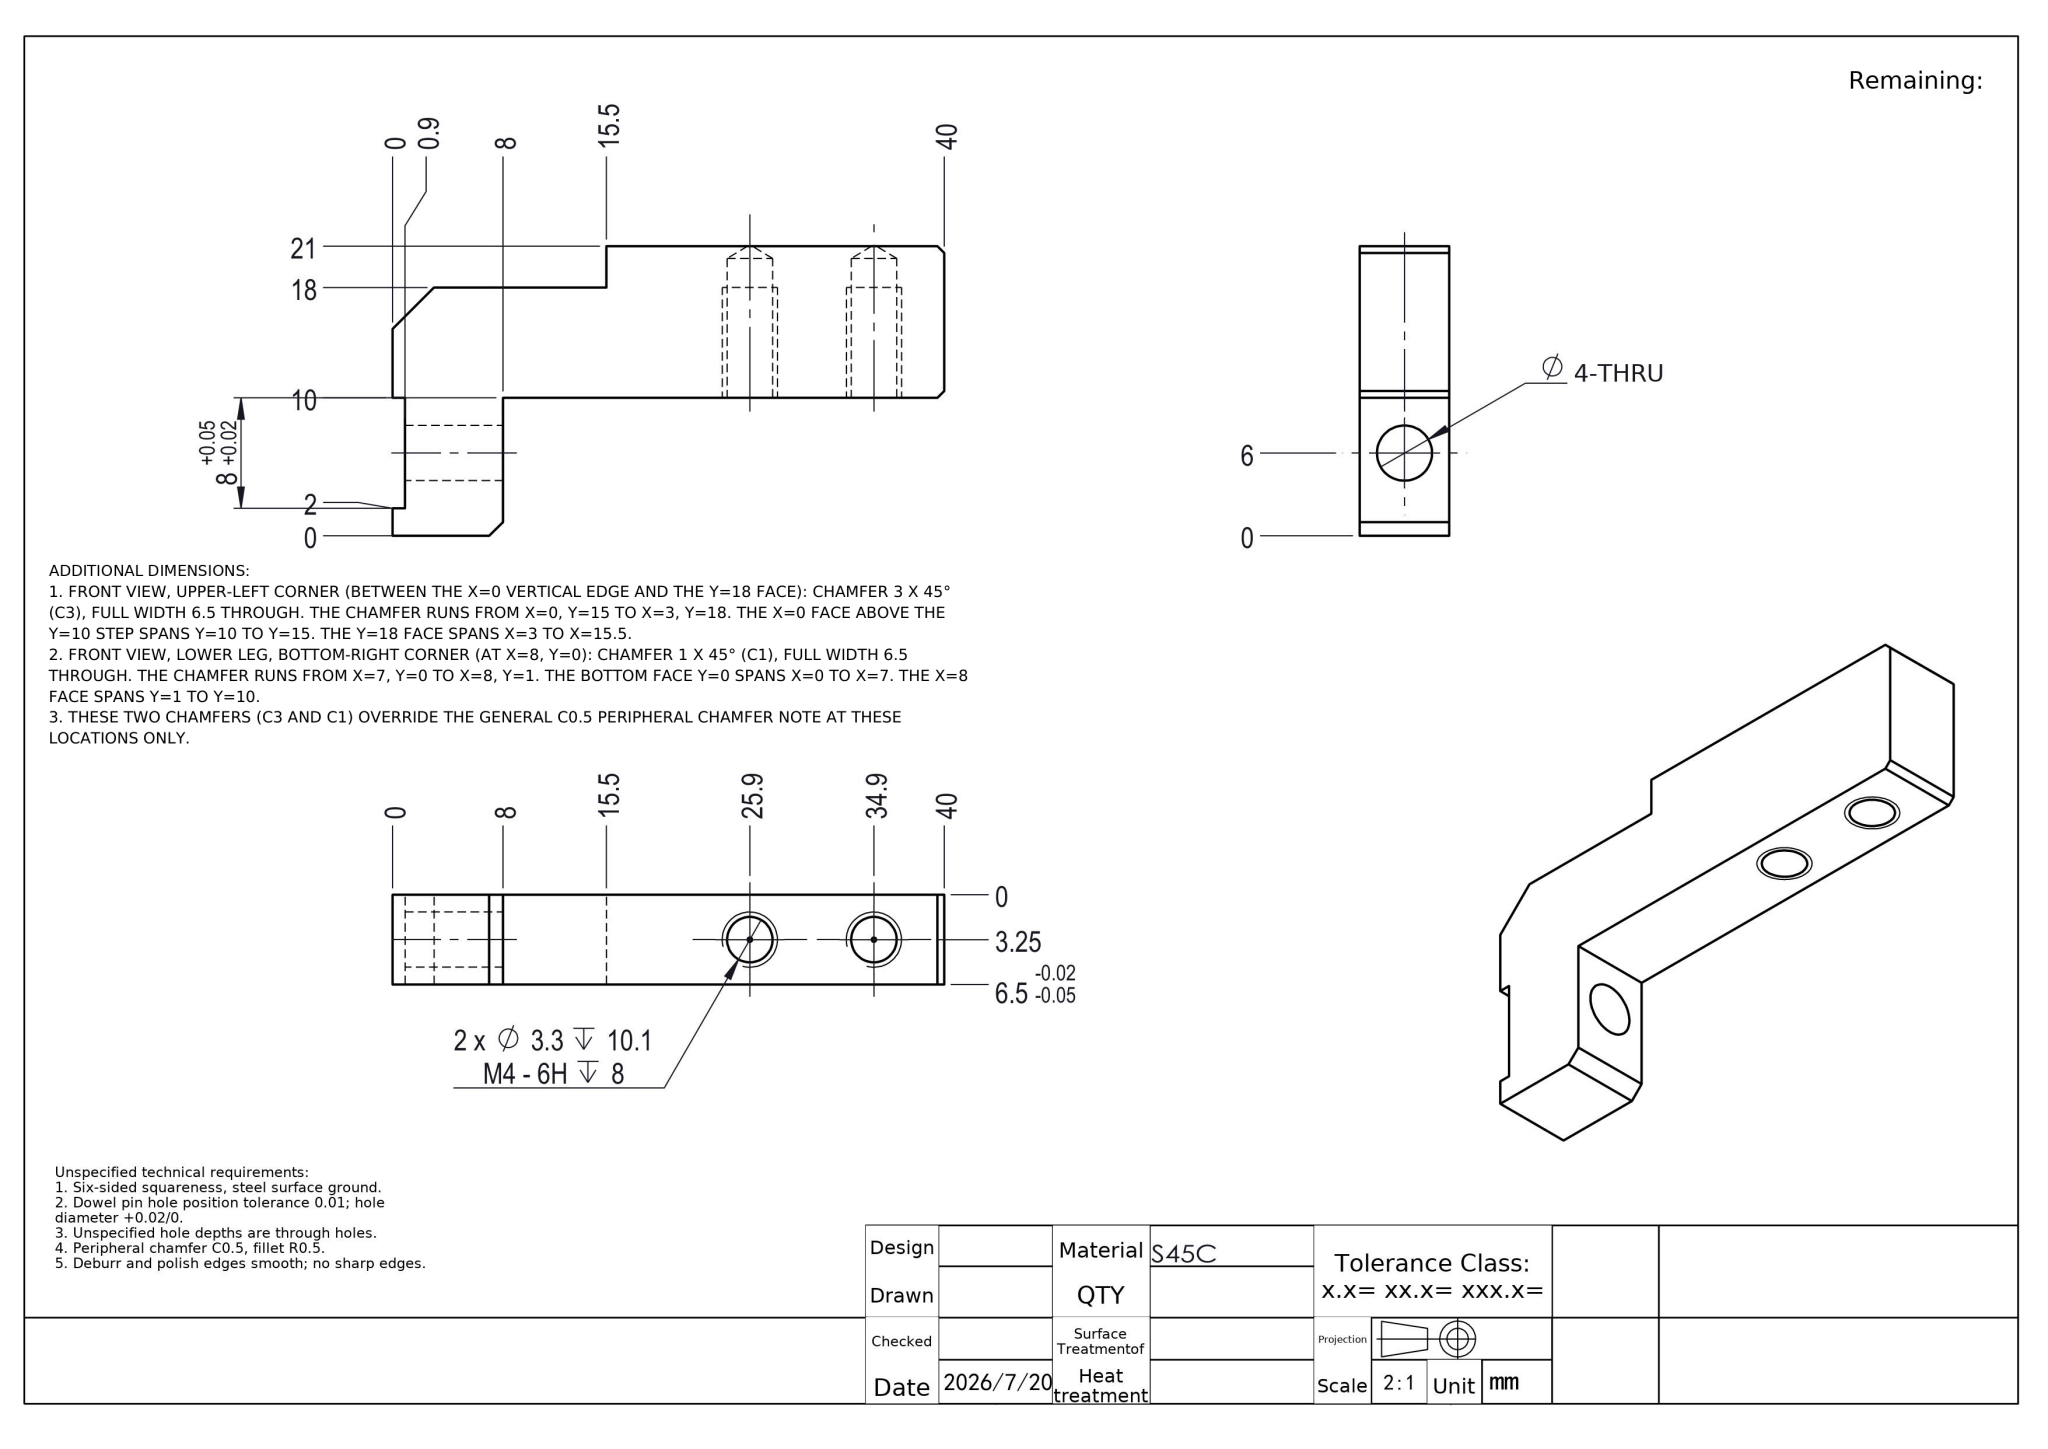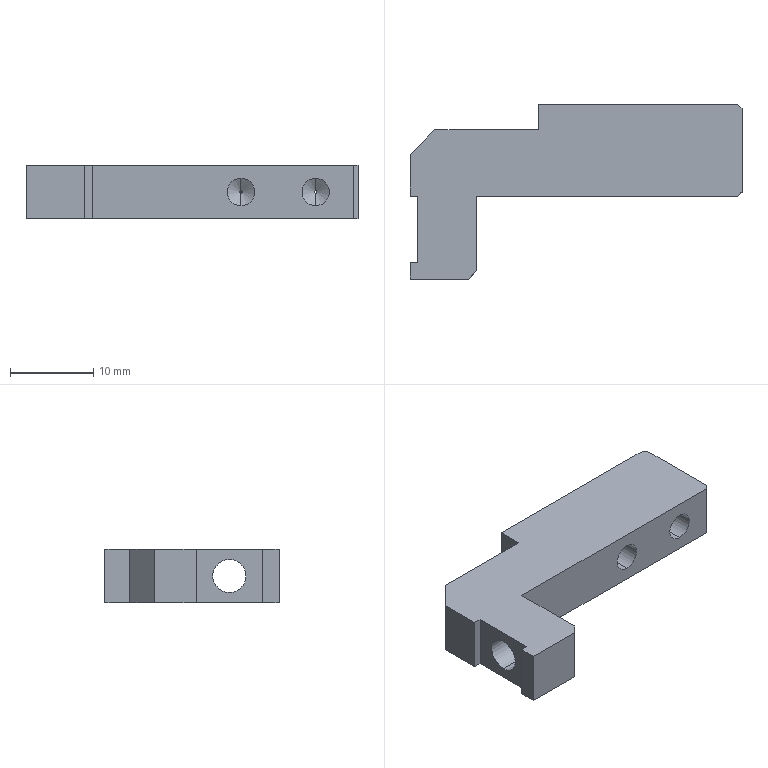Part | NX | mm | Stepped Three-Bore Angled Link Bracket | 1 solid | 28 faces | box 40 x 21 x 6.5 mm | volume 2729 mm3 | plane 18 | cylinder 6 | cone 4 | commonest cylinder face diameters 3.3 x4 4 x2
STEP:
#1=CARTESIAN_POINT('',(14.9,20.1,1.65));
#2=VERTEX_POINT('',#1);
#3=CARTESIAN_POINT('',(14.9,20.1,-1.65));
#4=VERTEX_POINT('',#3);
#5=CARTESIAN_POINT('',(14.9,20.1,0.));
#6=DIRECTION('',(0.,-1.,0.));
#7=DIRECTION('',(0.,0.,-1.));
#8=AXIS2_PLACEMENT_3D('',#5,#6,#7);
#9=CIRCLE('',#8,1.65);
#10=EDGE_CURVE('',#2,#4,#9,.T.);
#11=ORIENTED_EDGE('',*,*,#10,.F.);
#12=CARTESIAN_POINT('',(14.9,10.,1.65));
#13=VERTEX_POINT('',#12);
#14=CARTESIAN_POINT('',(14.9,10.,1.65));
#15=DIRECTION('',(0.,-1.,0.));
#16=VECTOR('',#15,1000.);
#17=LINE('',#14,#16);
#18=EDGE_CURVE('',#2,#13,#17,.T.);
#19=ORIENTED_EDGE('',*,*,#18,.T.);
#20=CARTESIAN_POINT('',(14.9,10.,-1.65));
#21=VERTEX_POINT('',#20);
#22=CARTESIAN_POINT('',(14.9,10.,0.));
#23=DIRECTION('',(0.,-1.,0.));
#24=DIRECTION('',(0.,0.,-1.));
#25=AXIS2_PLACEMENT_3D('',#22,#23,#24);
#26=CIRCLE('',#25,1.65);
#27=EDGE_CURVE('',#13,#21,#26,.T.);
#28=ORIENTED_EDGE('',*,*,#27,.T.);
#29=CARTESIAN_POINT('',(14.9,10.,-1.65));
#30=DIRECTION('',(0.,-1.,0.));
#31=VECTOR('',#30,1000.);
#32=LINE('',#29,#31);
#33=EDGE_CURVE('',#4,#21,#32,.T.);
#34=ORIENTED_EDGE('',*,*,#33,.F.);
#35=EDGE_LOOP('',(#11,#19,#28,#34));
#36=FACE_OUTER_BOUND('',#35,.T.);
#37=CARTESIAN_POINT('',(14.9,10.,0.));
#38=DIRECTION('',(0.,-1.,0.));
#39=DIRECTION('',(0.,0.,-1.));
#40=AXIS2_PLACEMENT_3D('',#37,#38,#39);
#41=CYLINDRICAL_SURFACE('',#40,1.65);
#42=ADVANCED_FACE('',(#36),#41,.F.);
#43=CARTESIAN_POINT('',(14.9,21.,-0.1521));
#44=VERTEX_POINT('',#43);
#45=CARTESIAN_POINT('',(14.9,21.,0.1521));
#46=VERTEX_POINT('',#45);
#47=CARTESIAN_POINT('',(14.9,21.,0.));
#48=DIRECTION('',(-0.,1.,0.));
#49=DIRECTION('',(-1.,0.,0.));
#50=AXIS2_PLACEMENT_3D('',#47,#48,#49);
#51=CIRCLE('',#50,0.1521);
#52=EDGE_CURVE('',#44,#46,#51,.T.);
#53=ORIENTED_EDGE('',*,*,#52,.T.);
#54=CARTESIAN_POINT('',(14.9,20.1,1.65));
#55=DIRECTION('',(0.,-0.515,0.8572));
#56=VECTOR('',#55,1000.);
#57=LINE('',#54,#56);
#58=EDGE_CURVE('',#46,#2,#57,.T.);
#59=ORIENTED_EDGE('',*,*,#58,.T.);
#60=ORIENTED_EDGE('',*,*,#10,.T.);
#61=CARTESIAN_POINT('',(14.9,20.1,-1.65));
#62=DIRECTION('',(0.,-0.515,-0.8572));
#63=VECTOR('',#62,1000.);
#64=LINE('',#61,#63);
#65=EDGE_CURVE('',#44,#4,#64,.T.);
#66=ORIENTED_EDGE('',*,*,#65,.F.);
#67=EDGE_LOOP('',(#53,#59,#60,#66));
#68=FACE_OUTER_BOUND('',#67,.T.);
#69=CARTESIAN_POINT('',(14.9,20.1,0.));
#70=DIRECTION('',(0.,-1.,0.));
#71=DIRECTION('',(0.,0.,-1.));
#72=AXIS2_PLACEMENT_3D('',#69,#70,#71);
#73=CONICAL_SURFACE('',#72,1.65,1.03);
#74=ADVANCED_FACE('',(#68),#73,.F.);
#75=CARTESIAN_POINT('',(5.9,20.1,1.65));
#76=VERTEX_POINT('',#75);
#77=CARTESIAN_POINT('',(5.9,20.1,-1.65));
#78=VERTEX_POINT('',#77);
#79=CARTESIAN_POINT('',(5.9,20.1,0.));
#80=DIRECTION('',(0.,-1.,0.));
#81=DIRECTION('',(0.,0.,-1.));
#82=AXIS2_PLACEMENT_3D('',#79,#80,#81);
#83=CIRCLE('',#82,1.65);
#84=EDGE_CURVE('',#76,#78,#83,.T.);
#85=ORIENTED_EDGE('',*,*,#84,.F.);
#86=CARTESIAN_POINT('',(5.9,10.,1.65));
#87=VERTEX_POINT('',#86);
#88=CARTESIAN_POINT('',(5.9,10.,1.65));
#89=DIRECTION('',(0.,-1.,0.));
#90=VECTOR('',#89,1000.);
#91=LINE('',#88,#90);
#92=EDGE_CURVE('',#76,#87,#91,.T.);
#93=ORIENTED_EDGE('',*,*,#92,.T.);
#94=CARTESIAN_POINT('',(5.9,10.,-1.65));
#95=VERTEX_POINT('',#94);
#96=CARTESIAN_POINT('',(5.9,10.,0.));
#97=DIRECTION('',(0.,-1.,0.));
#98=DIRECTION('',(0.,0.,-1.));
#99=AXIS2_PLACEMENT_3D('',#96,#97,#98);
#100=CIRCLE('',#99,1.65);
#101=EDGE_CURVE('',#87,#95,#100,.T.);
#102=ORIENTED_EDGE('',*,*,#101,.T.);
#103=CARTESIAN_POINT('',(5.9,10.,-1.65));
#104=DIRECTION('',(0.,-1.,0.));
#105=VECTOR('',#104,1000.);
#106=LINE('',#103,#105);
#107=EDGE_CURVE('',#78,#95,#106,.T.);
#108=ORIENTED_EDGE('',*,*,#107,.F.);
#109=EDGE_LOOP('',(#85,#93,#102,#108));
#110=FACE_OUTER_BOUND('',#109,.T.);
#111=CARTESIAN_POINT('',(5.9,10.,0.));
#112=DIRECTION('',(0.,-1.,0.));
#113=DIRECTION('',(0.,0.,-1.));
#114=AXIS2_PLACEMENT_3D('',#111,#112,#113);
#115=CYLINDRICAL_SURFACE('',#114,1.65);
#116=ADVANCED_FACE('',(#110),#115,.F.);
#117=CARTESIAN_POINT('',(5.9,21.,-0.1521));
#118=VERTEX_POINT('',#117);
#119=CARTESIAN_POINT('',(5.9,21.,0.1521));
#120=VERTEX_POINT('',#119);
#121=CARTESIAN_POINT('',(5.9,21.,0.));
#122=DIRECTION('',(-0.,1.,0.));
#123=DIRECTION('',(-1.,0.,0.));
#124=AXIS2_PLACEMENT_3D('',#121,#122,#123);
#125=CIRCLE('',#124,0.1521);
#126=EDGE_CURVE('',#118,#120,#125,.T.);
#127=ORIENTED_EDGE('',*,*,#126,.T.);
#128=CARTESIAN_POINT('',(5.9,20.1,1.65));
#129=DIRECTION('',(0.,-0.515,0.8572));
#130=VECTOR('',#129,1000.);
#131=LINE('',#128,#130);
#132=EDGE_CURVE('',#120,#76,#131,.T.);
#133=ORIENTED_EDGE('',*,*,#132,.T.);
#134=ORIENTED_EDGE('',*,*,#84,.T.);
#135=CARTESIAN_POINT('',(5.9,20.1,-1.65));
#136=DIRECTION('',(0.,-0.515,-0.8572));
#137=VECTOR('',#136,1000.);
#138=LINE('',#135,#137);
#139=EDGE_CURVE('',#118,#78,#138,.T.);
#140=ORIENTED_EDGE('',*,*,#139,.F.);
#141=EDGE_LOOP('',(#127,#133,#134,#140));
#142=FACE_OUTER_BOUND('',#141,.T.);
#143=CARTESIAN_POINT('',(5.9,20.1,0.));
#144=DIRECTION('',(0.,-1.,0.));
#145=DIRECTION('',(0.,0.,-1.));
#146=AXIS2_PLACEMENT_3D('',#143,#144,#145);
#147=CONICAL_SURFACE('',#146,1.65,1.03);
#148=ADVANCED_FACE('',(#142),#147,.F.);
#149=CARTESIAN_POINT('',(-19.1,6.,2.));
#150=VERTEX_POINT('',#149);
#151=CARTESIAN_POINT('',(-19.1,6.,-2.));
#152=VERTEX_POINT('',#151);
#153=CARTESIAN_POINT('',(-19.1,6.,0.));
#154=DIRECTION('',(1.,0.,0.));
#155=DIRECTION('',(0.,0.,-1.));
#156=AXIS2_PLACEMENT_3D('',#153,#154,#155);
#157=CIRCLE('',#156,2.);
#158=EDGE_CURVE('',#150,#152,#157,.T.);
#159=ORIENTED_EDGE('',*,*,#158,.F.);
#160=CARTESIAN_POINT('',(-12.,6.,2.));
#161=VERTEX_POINT('',#160);
#162=CARTESIAN_POINT('',(-20.,6.,2.));
#163=DIRECTION('',(1.,0.,0.));
#164=VECTOR('',#163,1000.);
#165=LINE('',#162,#164);
#166=EDGE_CURVE('',#150,#161,#165,.T.);
#167=ORIENTED_EDGE('',*,*,#166,.T.);
#168=CARTESIAN_POINT('',(-12.,6.,-2.));
#169=VERTEX_POINT('',#168);
#170=CARTESIAN_POINT('',(-12.,6.,0.));
#171=DIRECTION('',(1.,0.,0.));
#172=DIRECTION('',(0.,0.,-1.));
#173=AXIS2_PLACEMENT_3D('',#170,#171,#172);
#174=CIRCLE('',#173,2.);
#175=EDGE_CURVE('',#161,#169,#174,.T.);
#176=ORIENTED_EDGE('',*,*,#175,.T.);
#177=CARTESIAN_POINT('',(-20.,6.,-2.));
#178=DIRECTION('',(1.,0.,0.));
#179=VECTOR('',#178,1000.);
#180=LINE('',#177,#179);
#181=EDGE_CURVE('',#152,#169,#180,.T.);
#182=ORIENTED_EDGE('',*,*,#181,.F.);
#183=EDGE_LOOP('',(#159,#167,#176,#182));
#184=FACE_OUTER_BOUND('',#183,.T.);
#185=CARTESIAN_POINT('',(-20.,6.,0.));
#186=DIRECTION('',(1.,0.,0.));
#187=DIRECTION('',(0.,0.,-1.));
#188=AXIS2_PLACEMENT_3D('',#185,#186,#187);
#189=CYLINDRICAL_SURFACE('',#188,2.);
#190=ADVANCED_FACE('',(#184),#189,.F.);
#191=CARTESIAN_POINT('',(-20.,15.,3.25));
#192=VERTEX_POINT('',#191);
#193=CARTESIAN_POINT('',(-20.,10.,3.25));
#194=VERTEX_POINT('',#193);
#195=CARTESIAN_POINT('',(-20.,18.,3.25));
#196=DIRECTION('',(0.,-1.,0.));
#197=VECTOR('',#196,1000.);
#198=LINE('',#195,#197);
#199=EDGE_CURVE('',#192,#194,#198,.T.);
#200=ORIENTED_EDGE('',*,*,#199,.F.);
#201=CARTESIAN_POINT('',(-20.,15.,-3.25));
#202=VERTEX_POINT('',#201);
#203=CARTESIAN_POINT('',(-20.,15.,-3.25));
#204=DIRECTION('',(0.,0.,-1.));
#205=VECTOR('',#204,1000.);
#206=LINE('',#203,#205);
#207=EDGE_CURVE('',#192,#202,#206,.T.);
#208=ORIENTED_EDGE('',*,*,#207,.T.);
#209=CARTESIAN_POINT('',(-20.,10.,-3.25));
#210=VERTEX_POINT('',#209);
#211=CARTESIAN_POINT('',(-20.,18.,-3.25));
#212=DIRECTION('',(0.,-1.,0.));
#213=VECTOR('',#212,1000.);
#214=LINE('',#211,#213);
#215=EDGE_CURVE('',#202,#210,#214,.T.);
#216=ORIENTED_EDGE('',*,*,#215,.T.);
#217=CARTESIAN_POINT('',(-20.,10.,-3.25));
#218=DIRECTION('',(0.,0.,1.));
#219=VECTOR('',#218,1000.);
#220=LINE('',#217,#219);
#221=EDGE_CURVE('',#210,#194,#220,.T.);
#222=ORIENTED_EDGE('',*,*,#221,.T.);
#223=EDGE_LOOP('',(#200,#208,#216,#222));
#224=FACE_OUTER_BOUND('',#223,.T.);
#225=CARTESIAN_POINT('',(-20.,18.,-3.25));
#226=DIRECTION('',(1.,0.,0.));
#227=DIRECTION('',(0.,0.,-1.));
#228=AXIS2_PLACEMENT_3D('',#225,#226,#227);
#229=PLANE('',#228);
#230=ADVANCED_FACE('',(#224),#229,.F.);
#231=CARTESIAN_POINT('',(20.,20.5,-3.25));
#232=VERTEX_POINT('',#231);
#233=CARTESIAN_POINT('',(20.,10.5,-3.25));
#234=VERTEX_POINT('',#233);
#235=CARTESIAN_POINT('',(20.,18.,-3.25));
#236=DIRECTION('',(0.,-1.,0.));
#237=VECTOR('',#236,1000.);
#238=LINE('',#235,#237);
#239=EDGE_CURVE('',#232,#234,#238,.T.);
#240=ORIENTED_EDGE('',*,*,#239,.F.);
#241=CARTESIAN_POINT('',(20.,20.5,3.25));
#242=VERTEX_POINT('',#241);
#243=CARTESIAN_POINT('',(20.,20.5,3.25));
#244=DIRECTION('',(0.,0.,1.));
#245=VECTOR('',#244,1000.);
#246=LINE('',#243,#245);
#247=EDGE_CURVE('',#232,#242,#246,.T.);
#248=ORIENTED_EDGE('',*,*,#247,.T.);
#249=CARTESIAN_POINT('',(20.,10.5,3.25));
#250=VERTEX_POINT('',#249);
#251=CARTESIAN_POINT('',(20.,18.,3.25));
#252=DIRECTION('',(0.,-1.,0.));
#253=VECTOR('',#252,1000.);
#254=LINE('',#251,#253);
#255=EDGE_CURVE('',#242,#250,#254,.T.);
#256=ORIENTED_EDGE('',*,*,#255,.T.);
#257=CARTESIAN_POINT('',(20.,10.5,-3.25));
#258=DIRECTION('',(0.,0.,-1.));
#259=VECTOR('',#258,1000.);
#260=LINE('',#257,#259);
#261=EDGE_CURVE('',#250,#234,#260,.T.);
#262=ORIENTED_EDGE('',*,*,#261,.T.);
#263=EDGE_LOOP('',(#240,#248,#256,#262));
#264=FACE_OUTER_BOUND('',#263,.T.);
#265=CARTESIAN_POINT('',(20.,18.,-3.25));
#266=DIRECTION('',(-1.,0.,0.));
#267=DIRECTION('',(0.,0.,1.));
#268=AXIS2_PLACEMENT_3D('',#265,#266,#267);
#269=PLANE('',#268);
#270=ADVANCED_FACE('',(#264),#269,.F.);
#271=CARTESIAN_POINT('',(-4.5,21.,-3.25));
#272=VERTEX_POINT('',#271);
#273=CARTESIAN_POINT('',(19.5,21.,-3.25));
#274=VERTEX_POINT('',#273);
#275=CARTESIAN_POINT('',(20.,21.,-3.25));
#276=DIRECTION('',(1.,0.,0.));
#277=VECTOR('',#276,1000.);
#278=LINE('',#275,#277);
#279=EDGE_CURVE('',#272,#274,#278,.T.);
#280=ORIENTED_EDGE('',*,*,#279,.T.);
#281=CARTESIAN_POINT('',(20.,20.5,-3.25));
#282=DIRECTION('',(0.7071,-0.7071,0.));
#283=VECTOR('',#282,1000.);
#284=LINE('',#281,#283);
#285=EDGE_CURVE('',#274,#232,#284,.T.);
#286=ORIENTED_EDGE('',*,*,#285,.T.);
#287=ORIENTED_EDGE('',*,*,#239,.T.);
#288=CARTESIAN_POINT('',(19.5,10.,-3.25));
#289=VERTEX_POINT('',#288);
#290=CARTESIAN_POINT('',(20.,10.5,-3.25));
#291=DIRECTION('',(-0.7071,-0.7071,0.));
#292=VECTOR('',#291,1000.);
#293=LINE('',#290,#292);
#294=EDGE_CURVE('',#234,#289,#293,.T.);
#295=ORIENTED_EDGE('',*,*,#294,.T.);
#296=CARTESIAN_POINT('',(-12.,10.,-3.25));
#297=VERTEX_POINT('',#296);
#298=CARTESIAN_POINT('',(20.,10.,-3.25));
#299=DIRECTION('',(1.,0.,0.));
#300=VECTOR('',#299,1000.);
#301=LINE('',#298,#300);
#302=EDGE_CURVE('',#297,#289,#301,.T.);
#303=ORIENTED_EDGE('',*,*,#302,.F.);
#304=CARTESIAN_POINT('',(-12.,1.,-3.25));
#305=VERTEX_POINT('',#304);
#306=CARTESIAN_POINT('',(-12.,0.,-3.25));
#307=DIRECTION('',(0.,1.,0.));
#308=VECTOR('',#307,1000.);
#309=LINE('',#306,#308);
#310=EDGE_CURVE('',#305,#297,#309,.T.);
#311=ORIENTED_EDGE('',*,*,#310,.F.);
#312=CARTESIAN_POINT('',(-13.,0.,-3.25));
#313=VERTEX_POINT('',#312);
#314=CARTESIAN_POINT('',(-12.,1.,-3.25));
#315=DIRECTION('',(-0.7071,-0.7071,0.));
#316=VECTOR('',#315,1000.);
#317=LINE('',#314,#316);
#318=EDGE_CURVE('',#305,#313,#317,.T.);
#319=ORIENTED_EDGE('',*,*,#318,.T.);
#320=CARTESIAN_POINT('',(-20.,0.,-3.25));
#321=VERTEX_POINT('',#320);
#322=CARTESIAN_POINT('',(-20.,0.,-3.25));
#323=DIRECTION('',(-1.,0.,0.));
#324=VECTOR('',#323,1000.);
#325=LINE('',#322,#324);
#326=EDGE_CURVE('',#313,#321,#325,.T.);
#327=ORIENTED_EDGE('',*,*,#326,.T.);
#328=CARTESIAN_POINT('',(-20.,2.,-3.25));
#329=VERTEX_POINT('',#328);
#330=CARTESIAN_POINT('',(-20.,18.,-3.25));
#331=DIRECTION('',(0.,-1.,0.));
#332=VECTOR('',#331,1000.);
#333=LINE('',#330,#332);
#334=EDGE_CURVE('',#329,#321,#333,.T.);
#335=ORIENTED_EDGE('',*,*,#334,.F.);
#336=CARTESIAN_POINT('',(-19.1,2.,-3.25));
#337=VERTEX_POINT('',#336);
#338=CARTESIAN_POINT('',(-20.,2.,-3.25));
#339=DIRECTION('',(1.,0.,0.));
#340=VECTOR('',#339,1000.);
#341=LINE('',#338,#340);
#342=EDGE_CURVE('',#329,#337,#341,.T.);
#343=ORIENTED_EDGE('',*,*,#342,.T.);
#344=CARTESIAN_POINT('',(-19.1,10.,-3.25));
#345=VERTEX_POINT('',#344);
#346=CARTESIAN_POINT('',(-19.1,10.,-3.25));
#347=DIRECTION('',(0.,1.,0.));
#348=VECTOR('',#347,1000.);
#349=LINE('',#346,#348);
#350=EDGE_CURVE('',#337,#345,#349,.T.);
#351=ORIENTED_EDGE('',*,*,#350,.T.);
#352=CARTESIAN_POINT('',(-20.,10.,-3.25));
#353=DIRECTION('',(-1.,0.,0.));
#354=VECTOR('',#353,1000.);
#355=LINE('',#352,#354);
#356=EDGE_CURVE('',#345,#210,#355,.T.);
#357=ORIENTED_EDGE('',*,*,#356,.T.);
#358=ORIENTED_EDGE('',*,*,#215,.F.);
#359=CARTESIAN_POINT('',(-17.,18.,-3.25));
#360=VERTEX_POINT('',#359);
#361=CARTESIAN_POINT('',(-17.,18.,-3.25));
#362=DIRECTION('',(0.7071,0.7071,0.));
#363=VECTOR('',#362,1000.);
#364=LINE('',#361,#363);
#365=EDGE_CURVE('',#202,#360,#364,.T.);
#366=ORIENTED_EDGE('',*,*,#365,.T.);
#367=CARTESIAN_POINT('',(-4.5,18.,-3.25));
#368=VERTEX_POINT('',#367);
#369=CARTESIAN_POINT('',(-20.,18.,-3.25));
#370=DIRECTION('',(-1.,0.,0.));
#371=VECTOR('',#370,1000.);
#372=LINE('',#369,#371);
#373=EDGE_CURVE('',#368,#360,#372,.T.);
#374=ORIENTED_EDGE('',*,*,#373,.F.);
#375=CARTESIAN_POINT('',(-4.5,18.,-3.25));
#376=DIRECTION('',(0.,1.,0.));
#377=VECTOR('',#376,1000.);
#378=LINE('',#375,#377);
#379=EDGE_CURVE('',#368,#272,#378,.T.);
#380=ORIENTED_EDGE('',*,*,#379,.T.);
#381=EDGE_LOOP('',(#280,#286,#287,#295,#303,#311,#319,#327,#335,#343,#351,#357,#358,#366,#374,#380));
#382=FACE_OUTER_BOUND('',#381,.T.);
#383=CARTESIAN_POINT('',(-20.,18.,-3.25));
#384=DIRECTION('',(0.,0.,1.));
#385=DIRECTION('',(1.,0.,0.));
#386=AXIS2_PLACEMENT_3D('',#383,#384,#385);
#387=PLANE('',#386);
#388=ADVANCED_FACE('',(#382),#387,.F.);
#389=CARTESIAN_POINT('',(-20.,2.,3.25));
#390=VERTEX_POINT('',#389);
#391=CARTESIAN_POINT('',(-20.,0.,3.25));
#392=VERTEX_POINT('',#391);
#393=CARTESIAN_POINT('',(-20.,18.,3.25));
#394=DIRECTION('',(0.,-1.,0.));
#395=VECTOR('',#394,1000.);
#396=LINE('',#393,#395);
#397=EDGE_CURVE('',#390,#392,#396,.T.);
#398=ORIENTED_EDGE('',*,*,#397,.F.);
#399=CARTESIAN_POINT('',(-20.,2.,-3.25));
#400=DIRECTION('',(0.,0.,1.));
#401=VECTOR('',#400,1000.);
#402=LINE('',#399,#401);
#403=EDGE_CURVE('',#329,#390,#402,.T.);
#404=ORIENTED_EDGE('',*,*,#403,.F.);
#405=ORIENTED_EDGE('',*,*,#334,.T.);
#406=CARTESIAN_POINT('',(-20.,0.,-3.25));
#407=DIRECTION('',(0.,0.,1.));
#408=VECTOR('',#407,1000.);
#409=LINE('',#406,#408);
#410=EDGE_CURVE('',#321,#392,#409,.T.);
#411=ORIENTED_EDGE('',*,*,#410,.T.);
#412=EDGE_LOOP('',(#398,#404,#405,#411));
#413=FACE_OUTER_BOUND('',#412,.T.);
#414=CARTESIAN_POINT('',(-20.,18.,-3.25));
#415=DIRECTION('',(1.,0.,0.));
#416=DIRECTION('',(0.,0.,-1.));
#417=AXIS2_PLACEMENT_3D('',#414,#415,#416);
#418=PLANE('',#417);
#419=ADVANCED_FACE('',(#413),#418,.F.);
#420=ORIENTED_EDGE('',*,*,#255,.F.);
#421=CARTESIAN_POINT('',(19.5,21.,3.25));
#422=VERTEX_POINT('',#421);
#423=CARTESIAN_POINT('',(20.,20.5,3.25));
#424=DIRECTION('',(-0.7071,0.7071,0.));
#425=VECTOR('',#424,1000.);
#426=LINE('',#423,#425);
#427=EDGE_CURVE('',#242,#422,#426,.T.);
#428=ORIENTED_EDGE('',*,*,#427,.T.);
#429=CARTESIAN_POINT('',(-4.5,21.,3.25));
#430=VERTEX_POINT('',#429);
#431=CARTESIAN_POINT('',(20.,21.,3.25));
#432=DIRECTION('',(-1.,-0.,0.));
#433=VECTOR('',#432,1000.);
#434=LINE('',#431,#433);
#435=EDGE_CURVE('',#422,#430,#434,.T.);
#436=ORIENTED_EDGE('',*,*,#435,.T.);
#437=CARTESIAN_POINT('',(-4.5,18.,3.25));
#438=VERTEX_POINT('',#437);
#439=CARTESIAN_POINT('',(-4.5,18.,3.25));
#440=DIRECTION('',(0.,-1.,0.));
#441=VECTOR('',#440,1000.);
#442=LINE('',#439,#441);
#443=EDGE_CURVE('',#430,#438,#442,.T.);
#444=ORIENTED_EDGE('',*,*,#443,.T.);
#445=CARTESIAN_POINT('',(-17.,18.,3.25));
#446=VERTEX_POINT('',#445);
#447=CARTESIAN_POINT('',(-20.,18.,3.25));
#448=DIRECTION('',(1.,0.,0.));
#449=VECTOR('',#448,1000.);
#450=LINE('',#447,#449);
#451=EDGE_CURVE('',#446,#438,#450,.T.);
#452=ORIENTED_EDGE('',*,*,#451,.F.);
#453=CARTESIAN_POINT('',(-17.,18.,3.25));
#454=DIRECTION('',(-0.7071,-0.7071,0.));
#455=VECTOR('',#454,1000.);
#456=LINE('',#453,#455);
#457=EDGE_CURVE('',#446,#192,#456,.T.);
#458=ORIENTED_EDGE('',*,*,#457,.T.);
#459=ORIENTED_EDGE('',*,*,#199,.T.);
#460=CARTESIAN_POINT('',(-19.1,10.,3.25));
#461=VERTEX_POINT('',#460);
#462=CARTESIAN_POINT('',(-20.,10.,3.25));
#463=DIRECTION('',(-1.,0.,0.));
#464=VECTOR('',#463,1000.);
#465=LINE('',#462,#464);
#466=EDGE_CURVE('',#461,#194,#465,.T.);
#467=ORIENTED_EDGE('',*,*,#466,.F.);
#468=CARTESIAN_POINT('',(-19.1,2.,3.25));
#469=VERTEX_POINT('',#468);
#470=CARTESIAN_POINT('',(-19.1,10.,3.25));
#471=DIRECTION('',(0.,1.,0.));
#472=VECTOR('',#471,1000.);
#473=LINE('',#470,#472);
#474=EDGE_CURVE('',#469,#461,#473,.T.);
#475=ORIENTED_EDGE('',*,*,#474,.F.);
#476=CARTESIAN_POINT('',(-20.,2.,3.25));
#477=DIRECTION('',(1.,0.,0.));
#478=VECTOR('',#477,1000.);
#479=LINE('',#476,#478);
#480=EDGE_CURVE('',#390,#469,#479,.T.);
#481=ORIENTED_EDGE('',*,*,#480,.F.);
#482=ORIENTED_EDGE('',*,*,#397,.T.);
#483=CARTESIAN_POINT('',(-13.,0.,3.25));
#484=VERTEX_POINT('',#483);
#485=CARTESIAN_POINT('',(-20.,0.,3.25));
#486=DIRECTION('',(1.,0.,0.));
#487=VECTOR('',#486,1000.);
#488=LINE('',#485,#487);
#489=EDGE_CURVE('',#392,#484,#488,.T.);
#490=ORIENTED_EDGE('',*,*,#489,.T.);
#491=CARTESIAN_POINT('',(-12.,1.,3.25));
#492=VERTEX_POINT('',#491);
#493=CARTESIAN_POINT('',(-12.,1.,3.25));
#494=DIRECTION('',(0.7071,0.7071,0.));
#495=VECTOR('',#494,1000.);
#496=LINE('',#493,#495);
#497=EDGE_CURVE('',#484,#492,#496,.T.);
#498=ORIENTED_EDGE('',*,*,#497,.T.);
#499=CARTESIAN_POINT('',(-12.,10.,3.25));
#500=VERTEX_POINT('',#499);
#501=CARTESIAN_POINT('',(-12.,0.,3.25));
#502=DIRECTION('',(0.,1.,0.));
#503=VECTOR('',#502,1000.);
#504=LINE('',#501,#503);
#505=EDGE_CURVE('',#492,#500,#504,.T.);
#506=ORIENTED_EDGE('',*,*,#505,.T.);
#507=CARTESIAN_POINT('',(19.5,10.,3.25));
#508=VERTEX_POINT('',#507);
#509=CARTESIAN_POINT('',(20.,10.,3.25));
#510=DIRECTION('',(1.,0.,0.));
#511=VECTOR('',#510,1000.);
#512=LINE('',#509,#511);
#513=EDGE_CURVE('',#500,#508,#512,.T.);
#514=ORIENTED_EDGE('',*,*,#513,.T.);
#515=CARTESIAN_POINT('',(20.,10.5,3.25));
#516=DIRECTION('',(0.7071,0.7071,0.));
#517=VECTOR('',#516,1000.);
#518=LINE('',#515,#517);
#519=EDGE_CURVE('',#508,#250,#518,.T.);
#520=ORIENTED_EDGE('',*,*,#519,.T.);
#521=EDGE_LOOP('',(#420,#428,#436,#444,#452,#458,#459,#467,#475,#481,#482,#490,#498,#506,#514,#520));
#522=FACE_OUTER_BOUND('',#521,.T.);
#523=CARTESIAN_POINT('',(-20.,18.,3.25));
#524=DIRECTION('',(0.,0.,-1.));
#525=DIRECTION('',(-1.,0.,0.));
#526=AXIS2_PLACEMENT_3D('',#523,#524,#525);
#527=PLANE('',#526);
#528=ADVANCED_FACE('',(#522),#527,.F.);
#529=CARTESIAN_POINT('',(-4.5,18.,-27.933));
#530=DIRECTION('',(0.,0.,1.));
#531=VECTOR('',#530,1000.);
#532=LINE('',#529,#531);
#533=EDGE_CURVE('',#368,#438,#532,.T.);
#534=ORIENTED_EDGE('',*,*,#533,.F.);
#535=ORIENTED_EDGE('',*,*,#373,.T.);
#536=CARTESIAN_POINT('',(-17.,18.,3.25));
#537=DIRECTION('',(0.,0.,1.));
#538=VECTOR('',#537,1000.);
#539=LINE('',#536,#538);
#540=EDGE_CURVE('',#360,#446,#539,.T.);
#541=ORIENTED_EDGE('',*,*,#540,.T.);
#542=ORIENTED_EDGE('',*,*,#451,.T.);
#543=EDGE_LOOP('',(#534,#535,#541,#542));
#544=FACE_OUTER_BOUND('',#543,.T.);
#545=CARTESIAN_POINT('',(0.,18.,0.));
#546=DIRECTION('',(0.,1.,0.));
#547=DIRECTION('',(0.,0.,1.));
#548=AXIS2_PLACEMENT_3D('',#545,#546,#547);
#549=PLANE('',#548);
#550=ADVANCED_FACE('',(#544),#549,.T.);
#551=ORIENTED_EDGE('',*,*,#326,.F.);
#552=CARTESIAN_POINT('',(-13.,0.,0.));
#553=DIRECTION('',(0.,0.,1.));
#554=VECTOR('',#553,1000.);
#555=LINE('',#552,#554);
#556=EDGE_CURVE('',#313,#484,#555,.T.);
#557=ORIENTED_EDGE('',*,*,#556,.T.);
#558=ORIENTED_EDGE('',*,*,#489,.F.);
#559=ORIENTED_EDGE('',*,*,#410,.F.);
#560=EDGE_LOOP('',(#551,#557,#558,#559));
#561=FACE_OUTER_BOUND('',#560,.T.);
#562=CARTESIAN_POINT('',(0.,0.,0.));
#563=DIRECTION('',(0.,1.,0.));
#564=DIRECTION('',(0.,0.,1.));
#565=AXIS2_PLACEMENT_3D('',#562,#563,#564);
#566=PLANE('',#565);
#567=ADVANCED_FACE('',(#561),#566,.F.);
#568=CARTESIAN_POINT('',(14.9,10.,0.));
#569=DIRECTION('',(0.,-1.,0.));
#570=DIRECTION('',(0.,0.,-1.));
#571=AXIS2_PLACEMENT_3D('',#568,#569,#570);
#572=CIRCLE('',#571,1.65);
#573=EDGE_CURVE('',#21,#13,#572,.T.);
#574=ORIENTED_EDGE('',*,*,#573,.F.);
#575=ORIENTED_EDGE('',*,*,#27,.F.);
#576=EDGE_LOOP('',(#574,#575));
#577=FACE_BOUND('',#576,.T.);
#578=CARTESIAN_POINT('',(5.9,10.,0.));
#579=DIRECTION('',(0.,-1.,0.));
#580=DIRECTION('',(0.,0.,-1.));
#581=AXIS2_PLACEMENT_3D('',#578,#579,#580);
#582=CIRCLE('',#581,1.65);
#583=EDGE_CURVE('',#95,#87,#582,.T.);
#584=ORIENTED_EDGE('',*,*,#583,.F.);
#585=ORIENTED_EDGE('',*,*,#101,.F.);
#586=EDGE_LOOP('',(#584,#585));
#587=FACE_BOUND('',#586,.T.);
#588=ORIENTED_EDGE('',*,*,#302,.T.);
#589=CARTESIAN_POINT('',(19.5,10.,3.25));
#590=DIRECTION('',(0.,0.,1.));
#591=VECTOR('',#590,1000.);
#592=LINE('',#589,#591);
#593=EDGE_CURVE('',#289,#508,#592,.T.);
#594=ORIENTED_EDGE('',*,*,#593,.T.);
#595=ORIENTED_EDGE('',*,*,#513,.F.);
#596=CARTESIAN_POINT('',(-12.,10.,3.25));
#597=DIRECTION('',(0.,0.,-1.));
#598=VECTOR('',#597,1000.);
#599=LINE('',#596,#598);
#600=EDGE_CURVE('',#500,#297,#599,.T.);
#601=ORIENTED_EDGE('',*,*,#600,.T.);
#602=EDGE_LOOP('',(#588,#594,#595,#601));
#603=FACE_OUTER_BOUND('',#602,.T.);
#604=CARTESIAN_POINT('',(20.,10.,3.25));
#605=DIRECTION('',(0.,1.,0.));
#606=DIRECTION('',(0.,0.,1.));
#607=AXIS2_PLACEMENT_3D('',#604,#605,#606);
#608=PLANE('',#607);
#609=ADVANCED_FACE('',(#577,#587,#603),#608,.F.);
#610=CARTESIAN_POINT('',(-12.,6.,0.));
#611=DIRECTION('',(1.,0.,0.));
#612=DIRECTION('',(0.,0.,-1.));
#613=AXIS2_PLACEMENT_3D('',#610,#611,#612);
#614=CIRCLE('',#613,2.);
#615=EDGE_CURVE('',#169,#161,#614,.T.);
#616=ORIENTED_EDGE('',*,*,#615,.F.);
#617=ORIENTED_EDGE('',*,*,#175,.F.);
#618=EDGE_LOOP('',(#616,#617));
#619=FACE_BOUND('',#618,.T.);
#620=ORIENTED_EDGE('',*,*,#505,.F.);
#621=CARTESIAN_POINT('',(-12.,1.,3.25));
#622=DIRECTION('',(0.,0.,-1.));
#623=VECTOR('',#622,1000.);
#624=LINE('',#621,#623);
#625=EDGE_CURVE('',#492,#305,#624,.T.);
#626=ORIENTED_EDGE('',*,*,#625,.T.);
#627=ORIENTED_EDGE('',*,*,#310,.T.);
#628=ORIENTED_EDGE('',*,*,#600,.F.);
#629=EDGE_LOOP('',(#620,#626,#627,#628));
#630=FACE_OUTER_BOUND('',#629,.T.);
#631=CARTESIAN_POINT('',(-12.,0.,3.25));
#632=DIRECTION('',(-1.,0.,0.));
#633=DIRECTION('',(0.,0.,1.));
#634=AXIS2_PLACEMENT_3D('',#631,#632,#633);
#635=PLANE('',#634);
#636=ADVANCED_FACE('',(#619,#630),#635,.F.);
#637=ORIENTED_EDGE('',*,*,#466,.T.);
#638=ORIENTED_EDGE('',*,*,#221,.F.);
#639=ORIENTED_EDGE('',*,*,#356,.F.);
#640=CARTESIAN_POINT('',(-19.1,10.,-3.25));
#641=DIRECTION('',(0.,0.,1.));
#642=VECTOR('',#641,1000.);
#643=LINE('',#640,#642);
#644=EDGE_CURVE('',#345,#461,#643,.T.);
#645=ORIENTED_EDGE('',*,*,#644,.T.);
#646=EDGE_LOOP('',(#637,#638,#639,#645));
#647=FACE_OUTER_BOUND('',#646,.T.);
#648=CARTESIAN_POINT('',(-20.,10.,-3.25));
#649=DIRECTION('',(0.,1.,0.));
#650=DIRECTION('',(0.,0.,1.));
#651=AXIS2_PLACEMENT_3D('',#648,#649,#650);
#652=PLANE('',#651);
#653=ADVANCED_FACE('',(#647),#652,.F.);
#654=CARTESIAN_POINT('',(-19.1,6.,0.));
#655=DIRECTION('',(1.,0.,0.));
#656=DIRECTION('',(0.,0.,-1.));
#657=AXIS2_PLACEMENT_3D('',#654,#655,#656);
#658=CIRCLE('',#657,2.);
#659=EDGE_CURVE('',#152,#150,#658,.T.);
#660=ORIENTED_EDGE('',*,*,#659,.T.);
#661=ORIENTED_EDGE('',*,*,#158,.T.);
#662=EDGE_LOOP('',(#660,#661));
#663=FACE_BOUND('',#662,.T.);
#664=ORIENTED_EDGE('',*,*,#474,.T.);
#665=ORIENTED_EDGE('',*,*,#644,.F.);
#666=ORIENTED_EDGE('',*,*,#350,.F.);
#667=CARTESIAN_POINT('',(-19.1,2.,-3.25));
#668=DIRECTION('',(0.,0.,1.));
#669=VECTOR('',#668,1000.);
#670=LINE('',#667,#669);
#671=EDGE_CURVE('',#337,#469,#670,.T.);
#672=ORIENTED_EDGE('',*,*,#671,.T.);
#673=EDGE_LOOP('',(#664,#665,#666,#672));
#674=FACE_OUTER_BOUND('',#673,.T.);
#675=CARTESIAN_POINT('',(-19.1,10.,-3.25));
#676=DIRECTION('',(1.,0.,0.));
#677=DIRECTION('',(0.,0.,-1.));
#678=AXIS2_PLACEMENT_3D('',#675,#676,#677);
#679=PLANE('',#678);
#680=ADVANCED_FACE('',(#663,#674),#679,.F.);
#681=ORIENTED_EDGE('',*,*,#480,.T.);
#682=ORIENTED_EDGE('',*,*,#671,.F.);
#683=ORIENTED_EDGE('',*,*,#342,.F.);
#684=ORIENTED_EDGE('',*,*,#403,.T.);
#685=EDGE_LOOP('',(#681,#682,#683,#684));
#686=FACE_OUTER_BOUND('',#685,.T.);
#687=CARTESIAN_POINT('',(-20.,2.,-3.25));
#688=DIRECTION('',(0.,-1.,0.));
#689=DIRECTION('',(0.,0.,-1.));
#690=AXIS2_PLACEMENT_3D('',#687,#688,#689);
#691=PLANE('',#690);
#692=ADVANCED_FACE('',(#686),#691,.F.);
#693=ORIENTED_EDGE('',*,*,#166,.F.);
#694=ORIENTED_EDGE('',*,*,#659,.F.);
#695=ORIENTED_EDGE('',*,*,#181,.T.);
#696=ORIENTED_EDGE('',*,*,#615,.T.);
#697=EDGE_LOOP('',(#693,#694,#695,#696));
#698=FACE_OUTER_BOUND('',#697,.T.);
#699=CARTESIAN_POINT('',(-20.,6.,0.));
#700=DIRECTION('',(1.,0.,0.));
#701=DIRECTION('',(0.,0.,-1.));
#702=AXIS2_PLACEMENT_3D('',#699,#700,#701);
#703=CYLINDRICAL_SURFACE('',#702,2.);
#704=ADVANCED_FACE('',(#698),#703,.F.);
#705=ORIENTED_EDGE('',*,*,#365,.F.);
#706=ORIENTED_EDGE('',*,*,#207,.F.);
#707=ORIENTED_EDGE('',*,*,#457,.F.);
#708=ORIENTED_EDGE('',*,*,#540,.F.);
#709=EDGE_LOOP('',(#705,#706,#707,#708));
#710=FACE_OUTER_BOUND('',#709,.T.);
#711=CARTESIAN_POINT('',(-17.,18.,0.));
#712=DIRECTION('',(-0.7071,0.7071,0.));
#713=DIRECTION('',(0.,0.,-1.));
#714=AXIS2_PLACEMENT_3D('',#711,#712,#713);
#715=PLANE('',#714);
#716=ADVANCED_FACE('',(#710),#715,.T.);
#717=ORIENTED_EDGE('',*,*,#379,.F.);
#718=ORIENTED_EDGE('',*,*,#533,.T.);
#719=ORIENTED_EDGE('',*,*,#443,.F.);
#720=CARTESIAN_POINT('',(-4.5,21.,-27.933));
#721=DIRECTION('',(0.,0.,1.));
#722=VECTOR('',#721,1000.);
#723=LINE('',#720,#722);
#724=EDGE_CURVE('',#272,#430,#723,.T.);
#725=ORIENTED_EDGE('',*,*,#724,.F.);
#726=EDGE_LOOP('',(#717,#718,#719,#725));
#727=FACE_OUTER_BOUND('',#726,.T.);
#728=CARTESIAN_POINT('',(-4.5,18.,-27.933));
#729=DIRECTION('',(-1.,0.,0.));
#730=DIRECTION('',(0.,0.,1.));
#731=AXIS2_PLACEMENT_3D('',#728,#729,#730);
#732=PLANE('',#731);
#733=ADVANCED_FACE('',(#727),#732,.T.);
#734=ORIENTED_EDGE('',*,*,#52,.F.);
#735=CARTESIAN_POINT('',(14.9,21.,0.));
#736=DIRECTION('',(-0.,1.,0.));
#737=DIRECTION('',(-1.,0.,0.));
#738=AXIS2_PLACEMENT_3D('',#735,#736,#737);
#739=CIRCLE('',#738,0.1521);
#740=EDGE_CURVE('',#46,#44,#739,.T.);
#741=ORIENTED_EDGE('',*,*,#740,.F.);
#742=EDGE_LOOP('',(#734,#741));
#743=FACE_BOUND('',#742,.T.);
#744=ORIENTED_EDGE('',*,*,#126,.F.);
#745=CARTESIAN_POINT('',(5.9,21.,0.));
#746=DIRECTION('',(-0.,1.,0.));
#747=DIRECTION('',(-1.,0.,0.));
#748=AXIS2_PLACEMENT_3D('',#745,#746,#747);
#749=CIRCLE('',#748,0.1521);
#750=EDGE_CURVE('',#120,#118,#749,.T.);
#751=ORIENTED_EDGE('',*,*,#750,.F.);
#752=EDGE_LOOP('',(#744,#751));
#753=FACE_BOUND('',#752,.T.);
#754=ORIENTED_EDGE('',*,*,#435,.F.);
#755=CARTESIAN_POINT('',(19.5,21.,-3.25));
#756=DIRECTION('',(0.,0.,-1.));
#757=VECTOR('',#756,1000.);
#758=LINE('',#755,#757);
#759=EDGE_CURVE('',#422,#274,#758,.T.);
#760=ORIENTED_EDGE('',*,*,#759,.T.);
#761=ORIENTED_EDGE('',*,*,#279,.F.);
#762=ORIENTED_EDGE('',*,*,#724,.T.);
#763=EDGE_LOOP('',(#754,#760,#761,#762));
#764=FACE_OUTER_BOUND('',#763,.T.);
#765=CARTESIAN_POINT('',(20.,21.,-27.933));
#766=DIRECTION('',(-0.,1.,0.));
#767=DIRECTION('',(-1.,-0.,0.));
#768=AXIS2_PLACEMENT_3D('',#765,#766,#767);
#769=PLANE('',#768);
#770=ADVANCED_FACE('',(#743,#753,#764),#769,.T.);
#771=ORIENTED_EDGE('',*,*,#497,.F.);
#772=ORIENTED_EDGE('',*,*,#556,.F.);
#773=ORIENTED_EDGE('',*,*,#318,.F.);
#774=ORIENTED_EDGE('',*,*,#625,.F.);
#775=EDGE_LOOP('',(#771,#772,#773,#774));
#776=FACE_OUTER_BOUND('',#775,.T.);
#777=CARTESIAN_POINT('',(-12.,1.,3.25));
#778=DIRECTION('',(-0.7071,0.7071,0.));
#779=DIRECTION('',(0.,0.,-1.));
#780=AXIS2_PLACEMENT_3D('',#777,#778,#779);
#781=PLANE('',#780);
#782=ADVANCED_FACE('',(#776),#781,.F.);
#783=ORIENTED_EDGE('',*,*,#132,.F.);
#784=ORIENTED_EDGE('',*,*,#750,.T.);
#785=ORIENTED_EDGE('',*,*,#139,.T.);
#786=CARTESIAN_POINT('',(5.9,20.1,0.));
#787=DIRECTION('',(0.,-1.,0.));
#788=DIRECTION('',(0.,0.,-1.));
#789=AXIS2_PLACEMENT_3D('',#786,#787,#788);
#790=CIRCLE('',#789,1.65);
#791=EDGE_CURVE('',#78,#76,#790,.T.);
#792=ORIENTED_EDGE('',*,*,#791,.T.);
#793=EDGE_LOOP('',(#783,#784,#785,#792));
#794=FACE_OUTER_BOUND('',#793,.T.);
#795=CARTESIAN_POINT('',(5.9,20.1,0.));
#796=DIRECTION('',(0.,-1.,0.));
#797=DIRECTION('',(0.,0.,-1.));
#798=AXIS2_PLACEMENT_3D('',#795,#796,#797);
#799=CONICAL_SURFACE('',#798,1.65,1.03);
#800=ADVANCED_FACE('',(#794),#799,.F.);
#801=ORIENTED_EDGE('',*,*,#92,.F.);
#802=ORIENTED_EDGE('',*,*,#791,.F.);
#803=ORIENTED_EDGE('',*,*,#107,.T.);
#804=ORIENTED_EDGE('',*,*,#583,.T.);
#805=EDGE_LOOP('',(#801,#802,#803,#804));
#806=FACE_OUTER_BOUND('',#805,.T.);
#807=CARTESIAN_POINT('',(5.9,10.,0.));
#808=DIRECTION('',(0.,-1.,0.));
#809=DIRECTION('',(0.,0.,-1.));
#810=AXIS2_PLACEMENT_3D('',#807,#808,#809);
#811=CYLINDRICAL_SURFACE('',#810,1.65);
#812=ADVANCED_FACE('',(#806),#811,.F.);
#813=ORIENTED_EDGE('',*,*,#58,.F.);
#814=ORIENTED_EDGE('',*,*,#740,.T.);
#815=ORIENTED_EDGE('',*,*,#65,.T.);
#816=CARTESIAN_POINT('',(14.9,20.1,0.));
#817=DIRECTION('',(0.,-1.,0.));
#818=DIRECTION('',(0.,0.,-1.));
#819=AXIS2_PLACEMENT_3D('',#816,#817,#818);
#820=CIRCLE('',#819,1.65);
#821=EDGE_CURVE('',#4,#2,#820,.T.);
#822=ORIENTED_EDGE('',*,*,#821,.T.);
#823=EDGE_LOOP('',(#813,#814,#815,#822));
#824=FACE_OUTER_BOUND('',#823,.T.);
#825=CARTESIAN_POINT('',(14.9,20.1,0.));
#826=DIRECTION('',(0.,-1.,0.));
#827=DIRECTION('',(0.,0.,-1.));
#828=AXIS2_PLACEMENT_3D('',#825,#826,#827);
#829=CONICAL_SURFACE('',#828,1.65,1.03);
#830=ADVANCED_FACE('',(#824),#829,.F.);
#831=ORIENTED_EDGE('',*,*,#18,.F.);
#832=ORIENTED_EDGE('',*,*,#821,.F.);
#833=ORIENTED_EDGE('',*,*,#33,.T.);
#834=ORIENTED_EDGE('',*,*,#573,.T.);
#835=EDGE_LOOP('',(#831,#832,#833,#834));
#836=FACE_OUTER_BOUND('',#835,.T.);
#837=CARTESIAN_POINT('',(14.9,10.,0.));
#838=DIRECTION('',(0.,-1.,0.));
#839=DIRECTION('',(0.,0.,-1.));
#840=AXIS2_PLACEMENT_3D('',#837,#838,#839);
#841=CYLINDRICAL_SURFACE('',#840,1.65);
#842=ADVANCED_FACE('',(#836),#841,.F.);
#843=ORIENTED_EDGE('',*,*,#285,.F.);
#844=ORIENTED_EDGE('',*,*,#759,.F.);
#845=ORIENTED_EDGE('',*,*,#427,.F.);
#846=ORIENTED_EDGE('',*,*,#247,.F.);
#847=EDGE_LOOP('',(#843,#844,#845,#846));
#848=FACE_OUTER_BOUND('',#847,.T.);
#849=CARTESIAN_POINT('',(20.,20.5,-3.25));
#850=DIRECTION('',(0.7071,0.7071,0.));
#851=DIRECTION('',(0.,0.,-1.));
#852=AXIS2_PLACEMENT_3D('',#849,#850,#851);
#853=PLANE('',#852);
#854=ADVANCED_FACE('',(#848),#853,.T.);
#855=ORIENTED_EDGE('',*,*,#519,.F.);
#856=ORIENTED_EDGE('',*,*,#593,.F.);
#857=ORIENTED_EDGE('',*,*,#294,.F.);
#858=ORIENTED_EDGE('',*,*,#261,.F.);
#859=EDGE_LOOP('',(#855,#856,#857,#858));
#860=FACE_OUTER_BOUND('',#859,.T.);
#861=CARTESIAN_POINT('',(20.,10.5,-3.25));
#862=DIRECTION('',(-0.7071,0.7071,0.));
#863=DIRECTION('',(0.,0.,-1.));
#864=AXIS2_PLACEMENT_3D('',#861,#862,#863);
#865=PLANE('',#864);
#866=ADVANCED_FACE('',(#860),#865,.F.);
#867=CLOSED_SHELL('',(#42,#74,#116,#148,#190,#230,#270,#388,#419,#528,#550,#567,#609,#636,#653,#680,#692,#704,#716,#733,#770,#782,#800,#812,#830,#842,#854,#866));
#868=MANIFOLD_SOLID_BREP('',#867);
#869=CARTESIAN_POINT('',(0.,0.,0.));
#870=DIRECTION('',(0.,0.,1.));
#871=DIRECTION('',(1.,0.,0.));
#872=AXIS2_PLACEMENT_3D('',#869,#870,#871);
#873=(LENGTH_UNIT()NAMED_UNIT(*)SI_UNIT(.MILLI.,.METRE.));
#874=UNCERTAINTY_MEASURE_WITH_UNIT(LENGTH_MEASURE(0.00001),#873,'','');
#875=(NAMED_UNIT(*)PLANE_ANGLE_UNIT()SI_UNIT($,.RADIAN.));
#876=(NAMED_UNIT(*)SI_UNIT($,.STERADIAN.)SOLID_ANGLE_UNIT());
#877=(GEOMETRIC_REPRESENTATION_CONTEXT(3)GLOBAL_UNCERTAINTY_ASSIGNED_CONTEXT((#874))GLOBAL_UNIT_ASSIGNED_CONTEXT((#873,#875,#876))REPRESENTATION_CONTEXT('',''));
#878=ADVANCED_BREP_SHAPE_REPRESENTATION('',(#868,#872),#877);
#879=COLOUR_RGB('',0.7922,0.8196,0.9333);
#880=FILL_AREA_STYLE_COLOUR('',#879);
#881=FILL_AREA_STYLE('',(#880));
#882=SURFACE_STYLE_FILL_AREA(#881);
#883=SURFACE_SIDE_STYLE('',(#882));
#884=SURFACE_STYLE_USAGE(.BOTH.,#883);
#885=PRESENTATION_STYLE_ASSIGNMENT((#884));
#886=STYLED_ITEM('',(#885),#868);
#887=(LENGTH_UNIT()NAMED_UNIT(*)SI_UNIT(.MILLI.,.METRE.));
#888=UNCERTAINTY_MEASURE_WITH_UNIT(LENGTH_MEASURE(0.00001),#887,'','');
#889=(NAMED_UNIT(*)PLANE_ANGLE_UNIT()SI_UNIT($,.RADIAN.));
#890=(NAMED_UNIT(*)SI_UNIT($,.STERADIAN.)SOLID_ANGLE_UNIT());
#891=(GEOMETRIC_REPRESENTATION_CONTEXT(3)GLOBAL_UNCERTAINTY_ASSIGNED_CONTEXT((#888))GLOBAL_UNIT_ASSIGNED_CONTEXT((#887,#889,#890))REPRESENTATION_CONTEXT('',''));
#892=MECHANICAL_DESIGN_GEOMETRIC_PRESENTATION_REPRESENTATION('',(#886),#891);
#893=PRESENTATION_LAYER_ASSIGNMENT('','',(#886));